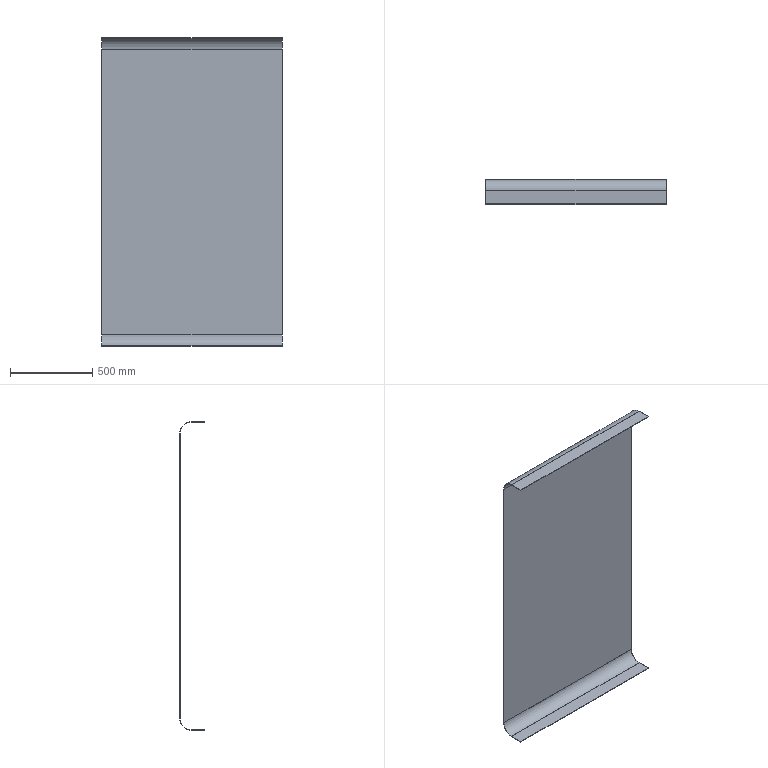Component | SolidWorks | TopHousingAssembly-1_CasingB-1 | 1 solid | 22 faces | box 1100 x 149.5 x 1881 mm | volume 6981573 mm3 | plane 18 | cylinder 4 | commonest cylinder face diameters 139 x2 133 x2
STEP:
#1=CARTESIAN_POINT('',(0.,96.791,2.618));
#2=VERTEX_POINT('',#1);
#3=CARTESIAN_POINT('',(0.,96.909,2.618));
#4=VERTEX_POINT('',#3);
#5=CARTESIAN_POINT('',(0.,96.909,2.618));
#6=DIRECTION('',(0.,1.,0.));
#7=VECTOR('',#6,39.37);
#8=LINE('',#5,#7);
#9=EDGE_CURVE('',#2,#4,#8,.T.);
#10=ORIENTED_EDGE('',*,*,#9,.F.);
#11=CARTESIAN_POINT('',(0.,96.791,71.201));
#12=VERTEX_POINT('',#11);
#13=CARTESIAN_POINT('',(0.,96.791,36.909));
#14=DIRECTION('',(0.,0.,1.));
#15=VECTOR('',#14,39.37);
#16=LINE('',#13,#15);
#17=EDGE_CURVE('',#2,#12,#16,.T.);
#18=ORIENTED_EDGE('',*,*,#17,.T.);
#19=CARTESIAN_POINT('',(0.,96.909,71.201));
#20=VERTEX_POINT('',#19);
#21=CARTESIAN_POINT('',(0.,96.909,71.201));
#22=DIRECTION('',(0.,1.,0.));
#23=VECTOR('',#22,39.37);
#24=LINE('',#21,#23);
#25=EDGE_CURVE('',#12,#20,#24,.T.);
#26=ORIENTED_EDGE('',*,*,#25,.T.);
#27=CARTESIAN_POINT('',(0.,96.909,71.201));
#28=DIRECTION('',(0.,0.,1.));
#29=VECTOR('',#28,39.37);
#30=LINE('',#27,#29);
#31=EDGE_CURVE('',#4,#20,#30,.T.);
#32=ORIENTED_EDGE('',*,*,#31,.F.);
#33=EDGE_LOOP('',(#10,#18,#26,#32));
#34=FACE_OUTER_BOUND('',#33,.T.);
#35=CARTESIAN_POINT('',(0.,96.909,71.201));
#36=DIRECTION('',(1.,0.,0.));
#37=DIRECTION('',(0.,0.,1.));
#38=AXIS2_PLACEMENT_3D('',#35,#36,#37);
#39=PLANE('',#38);
#40=ADVANCED_FACE('',(#34),#39,.F.);
#41=CARTESIAN_POINT('',(43.307,96.791,71.201));
#42=VERTEX_POINT('',#41);
#43=CARTESIAN_POINT('',(43.307,96.909,71.201));
#44=VERTEX_POINT('',#43);
#45=CARTESIAN_POINT('',(43.307,96.909,71.201));
#46=DIRECTION('',(0.,1.,0.));
#47=VECTOR('',#46,39.37);
#48=LINE('',#45,#47);
#49=EDGE_CURVE('',#42,#44,#48,.T.);
#50=ORIENTED_EDGE('',*,*,#49,.F.);
#51=CARTESIAN_POINT('',(43.307,96.791,2.618));
#52=VERTEX_POINT('',#51);
#53=CARTESIAN_POINT('',(43.307,96.791,36.909));
#54=DIRECTION('',(0.,0.,-1.));
#55=VECTOR('',#54,39.37);
#56=LINE('',#53,#55);
#57=EDGE_CURVE('',#42,#52,#56,.T.);
#58=ORIENTED_EDGE('',*,*,#57,.T.);
#59=CARTESIAN_POINT('',(43.307,96.909,2.618));
#60=VERTEX_POINT('',#59);
#61=CARTESIAN_POINT('',(43.307,96.909,2.618));
#62=DIRECTION('',(0.,1.,0.));
#63=VECTOR('',#62,39.37);
#64=LINE('',#61,#63);
#65=EDGE_CURVE('',#52,#60,#64,.T.);
#66=ORIENTED_EDGE('',*,*,#65,.T.);
#67=CARTESIAN_POINT('',(43.307,96.909,71.201));
#68=DIRECTION('',(0.,0.,-1.));
#69=VECTOR('',#68,39.37);
#70=LINE('',#67,#69);
#71=EDGE_CURVE('',#44,#60,#70,.T.);
#72=ORIENTED_EDGE('',*,*,#71,.F.);
#73=EDGE_LOOP('',(#50,#58,#66,#72));
#74=FACE_OUTER_BOUND('',#73,.T.);
#75=CARTESIAN_POINT('',(43.307,96.909,71.201));
#76=DIRECTION('',(-1.,0.,0.));
#77=DIRECTION('',(0.,0.,-1.));
#78=AXIS2_PLACEMENT_3D('',#75,#76,#77);
#79=PLANE('',#78);
#80=ADVANCED_FACE('',(#74),#79,.F.);
#81=ORIENTED_EDGE('',*,*,#71,.T.);
#82=CARTESIAN_POINT('',(0.,96.909,2.618));
#83=DIRECTION('',(-1.,0.,0.));
#84=VECTOR('',#83,39.37);
#85=LINE('',#82,#84);
#86=EDGE_CURVE('',#60,#4,#85,.T.);
#87=ORIENTED_EDGE('',*,*,#86,.T.);
#88=ORIENTED_EDGE('',*,*,#31,.T.);
#89=CARTESIAN_POINT('',(0.,96.909,71.201));
#90=DIRECTION('',(1.,0.,0.));
#91=VECTOR('',#90,39.37);
#92=LINE('',#89,#91);
#93=EDGE_CURVE('',#20,#44,#92,.T.);
#94=ORIENTED_EDGE('',*,*,#93,.T.);
#95=EDGE_LOOP('',(#81,#87,#88,#94));
#96=FACE_OUTER_BOUND('',#95,.T.);
#97=CARTESIAN_POINT('',(21.654,96.909,36.909));
#98=DIRECTION('',(0.,-1.,0.));
#99=DIRECTION('',(0.,0.,-1.));
#100=AXIS2_PLACEMENT_3D('',#97,#98,#99);
#101=PLANE('',#100);
#102=ADVANCED_FACE('',(#96),#101,.F.);
#103=ORIENTED_EDGE('',*,*,#57,.F.);
#104=CARTESIAN_POINT('',(21.654,96.791,71.201));
#105=DIRECTION('',(1.,0.,0.));
#106=VECTOR('',#105,39.37);
#107=LINE('',#104,#106);
#108=EDGE_CURVE('',#12,#42,#107,.T.);
#109=ORIENTED_EDGE('',*,*,#108,.F.);
#110=ORIENTED_EDGE('',*,*,#17,.F.);
#111=CARTESIAN_POINT('',(21.654,96.791,2.618));
#112=DIRECTION('',(-1.,0.,0.));
#113=VECTOR('',#112,39.37);
#114=LINE('',#111,#113);
#115=EDGE_CURVE('',#52,#2,#114,.T.);
#116=ORIENTED_EDGE('',*,*,#115,.F.);
#117=EDGE_LOOP('',(#103,#109,#110,#116));
#118=FACE_OUTER_BOUND('',#117,.T.);
#119=CARTESIAN_POINT('',(21.654,96.791,36.909));
#120=DIRECTION('',(0.,-1.,0.));
#121=DIRECTION('',(0.,0.,-1.));
#122=AXIS2_PLACEMENT_3D('',#119,#120,#121);
#123=PLANE('',#122);
#124=ADVANCED_FACE('',(#118),#123,.T.);
#125=CARTESIAN_POINT('',(43.307,94.173,73.819));
#126=VERTEX_POINT('',#125);
#127=CARTESIAN_POINT('',(43.307,94.173,73.937));
#128=VERTEX_POINT('',#127);
#129=CARTESIAN_POINT('',(43.307,94.173,73.937));
#130=DIRECTION('',(0.,0.,1.));
#131=VECTOR('',#130,39.37);
#132=LINE('',#129,#131);
#133=EDGE_CURVE('',#126,#128,#132,.T.);
#134=ORIENTED_EDGE('',*,*,#133,.F.);
#135=CARTESIAN_POINT('',(43.307,94.173,71.201));
#136=DIRECTION('',(1.,0.,0.));
#137=DIRECTION('',(0.,-0.,1.));
#138=AXIS2_PLACEMENT_3D('',#135,#136,#137);
#139=CIRCLE('',#138,2.618);
#140=EDGE_CURVE('',#42,#126,#139,.T.);
#141=ORIENTED_EDGE('',*,*,#140,.F.);
#142=ORIENTED_EDGE('',*,*,#49,.T.);
#143=CARTESIAN_POINT('',(43.307,94.173,71.201));
#144=DIRECTION('',(1.,0.,0.));
#145=DIRECTION('',(0.,-0.,1.));
#146=AXIS2_PLACEMENT_3D('',#143,#144,#145);
#147=CIRCLE('',#146,2.736);
#148=EDGE_CURVE('',#44,#128,#147,.T.);
#149=ORIENTED_EDGE('',*,*,#148,.T.);
#150=EDGE_LOOP('',(#134,#141,#142,#149));
#151=FACE_OUTER_BOUND('',#150,.T.);
#152=CARTESIAN_POINT('',(43.307,94.173,71.201));
#153=DIRECTION('',(1.,0.,0.));
#154=DIRECTION('',(0.,0.,-1.));
#155=AXIS2_PLACEMENT_3D('',#152,#153,#154);
#156=PLANE('',#155);
#157=ADVANCED_FACE('',(#151),#156,.T.);
#158=CARTESIAN_POINT('',(0.,94.173,73.819));
#159=VERTEX_POINT('',#158);
#160=CARTESIAN_POINT('',(0.,94.173,71.201));
#161=DIRECTION('',(-1.,0.,0.));
#162=DIRECTION('',(0.,0.,1.));
#163=AXIS2_PLACEMENT_3D('',#160,#161,#162);
#164=CIRCLE('',#163,2.618);
#165=EDGE_CURVE('',#159,#12,#164,.T.);
#166=ORIENTED_EDGE('',*,*,#165,.F.);
#167=CARTESIAN_POINT('',(0.,94.173,73.937));
#168=VERTEX_POINT('',#167);
#169=CARTESIAN_POINT('',(0.,94.173,73.819));
#170=DIRECTION('',(0.,0.,1.));
#171=VECTOR('',#170,39.37);
#172=LINE('',#169,#171);
#173=EDGE_CURVE('',#159,#168,#172,.T.);
#174=ORIENTED_EDGE('',*,*,#173,.T.);
#175=CARTESIAN_POINT('',(0.,94.173,71.201));
#176=DIRECTION('',(-1.,0.,0.));
#177=DIRECTION('',(0.,0.,1.));
#178=AXIS2_PLACEMENT_3D('',#175,#176,#177);
#179=CIRCLE('',#178,2.736);
#180=EDGE_CURVE('',#168,#20,#179,.T.);
#181=ORIENTED_EDGE('',*,*,#180,.T.);
#182=ORIENTED_EDGE('',*,*,#25,.F.);
#183=EDGE_LOOP('',(#166,#174,#181,#182));
#184=FACE_OUTER_BOUND('',#183,.T.);
#185=CARTESIAN_POINT('',(0.,94.173,71.201));
#186=DIRECTION('',(1.,0.,0.));
#187=DIRECTION('',(0.,0.,-1.));
#188=AXIS2_PLACEMENT_3D('',#185,#186,#187);
#189=PLANE('',#188);
#190=ADVANCED_FACE('',(#184),#189,.F.);
#191=ORIENTED_EDGE('',*,*,#93,.F.);
#192=ORIENTED_EDGE('',*,*,#180,.F.);
#193=CARTESIAN_POINT('',(43.307,94.173,73.937));
#194=DIRECTION('',(1.,0.,0.));
#195=VECTOR('',#194,39.37);
#196=LINE('',#193,#195);
#197=EDGE_CURVE('',#168,#128,#196,.T.);
#198=ORIENTED_EDGE('',*,*,#197,.T.);
#199=ORIENTED_EDGE('',*,*,#148,.F.);
#200=EDGE_LOOP('',(#191,#192,#198,#199));
#201=FACE_OUTER_BOUND('',#200,.T.);
#202=CARTESIAN_POINT('',(0.,94.173,71.201));
#203=DIRECTION('',(-1.,0.,0.));
#204=DIRECTION('',(0.,0.,1.));
#205=AXIS2_PLACEMENT_3D('',#202,#203,#204);
#206=CYLINDRICAL_SURFACE('',#205,2.736);
#207=ADVANCED_FACE('',(#201),#206,.T.);
#208=ORIENTED_EDGE('',*,*,#108,.T.);
#209=ORIENTED_EDGE('',*,*,#140,.T.);
#210=CARTESIAN_POINT('',(43.307,94.173,73.819));
#211=DIRECTION('',(-1.,0.,0.));
#212=VECTOR('',#211,39.37);
#213=LINE('',#210,#212);
#214=EDGE_CURVE('',#126,#159,#213,.T.);
#215=ORIENTED_EDGE('',*,*,#214,.T.);
#216=ORIENTED_EDGE('',*,*,#165,.T.);
#217=EDGE_LOOP('',(#208,#209,#215,#216));
#218=FACE_OUTER_BOUND('',#217,.T.);
#219=CARTESIAN_POINT('',(0.,94.173,71.201));
#220=DIRECTION('',(-1.,0.,0.));
#221=DIRECTION('',(0.,0.,1.));
#222=AXIS2_PLACEMENT_3D('',#219,#220,#221);
#223=CYLINDRICAL_SURFACE('',#222,2.618);
#224=ADVANCED_FACE('',(#218),#223,.F.);
#225=ORIENTED_EDGE('',*,*,#173,.F.);
#226=CARTESIAN_POINT('',(0.,91.024,73.819));
#227=VERTEX_POINT('',#226);
#228=CARTESIAN_POINT('',(0.,91.024,73.819));
#229=DIRECTION('',(0.,-1.,0.));
#230=VECTOR('',#229,39.37);
#231=LINE('',#228,#230);
#232=EDGE_CURVE('',#159,#227,#231,.T.);
#233=ORIENTED_EDGE('',*,*,#232,.T.);
#234=CARTESIAN_POINT('',(0.,91.024,73.937));
#235=VERTEX_POINT('',#234);
#236=CARTESIAN_POINT('',(0.,91.024,73.937));
#237=DIRECTION('',(0.,-0.,-1.));
#238=VECTOR('',#237,39.37);
#239=LINE('',#236,#238);
#240=EDGE_CURVE('',#235,#227,#239,.T.);
#241=ORIENTED_EDGE('',*,*,#240,.F.);
#242=CARTESIAN_POINT('',(0.,96.791,73.937));
#243=DIRECTION('',(0.,-1.,0.));
#244=VECTOR('',#243,39.37);
#245=LINE('',#242,#244);
#246=EDGE_CURVE('',#168,#235,#245,.T.);
#247=ORIENTED_EDGE('',*,*,#246,.F.);
#248=EDGE_LOOP('',(#225,#233,#241,#247));
#249=FACE_OUTER_BOUND('',#248,.T.);
#250=CARTESIAN_POINT('',(0.,91.024,73.937));
#251=DIRECTION('',(1.,0.,-0.));
#252=DIRECTION('',(-0.,1.,0.));
#253=AXIS2_PLACEMENT_3D('',#250,#251,#252);
#254=PLANE('',#253);
#255=ADVANCED_FACE('',(#249),#254,.F.);
#256=ORIENTED_EDGE('',*,*,#133,.T.);
#257=CARTESIAN_POINT('',(43.307,91.024,73.937));
#258=VERTEX_POINT('',#257);
#259=CARTESIAN_POINT('',(43.307,96.791,73.937));
#260=DIRECTION('',(0.,1.,-0.));
#261=VECTOR('',#260,39.37);
#262=LINE('',#259,#261);
#263=EDGE_CURVE('',#258,#128,#262,.T.);
#264=ORIENTED_EDGE('',*,*,#263,.F.);
#265=CARTESIAN_POINT('',(43.307,91.024,73.819));
#266=VERTEX_POINT('',#265);
#267=CARTESIAN_POINT('',(43.307,91.024,73.937));
#268=DIRECTION('',(0.,-0.,-1.));
#269=VECTOR('',#268,39.37);
#270=LINE('',#267,#269);
#271=EDGE_CURVE('',#258,#266,#270,.T.);
#272=ORIENTED_EDGE('',*,*,#271,.T.);
#273=CARTESIAN_POINT('',(43.307,96.791,73.819));
#274=DIRECTION('',(0.,1.,-0.));
#275=VECTOR('',#274,39.37);
#276=LINE('',#273,#275);
#277=EDGE_CURVE('',#266,#126,#276,.T.);
#278=ORIENTED_EDGE('',*,*,#277,.T.);
#279=EDGE_LOOP('',(#256,#264,#272,#278));
#280=FACE_OUTER_BOUND('',#279,.T.);
#281=CARTESIAN_POINT('',(43.307,96.791,73.937));
#282=DIRECTION('',(-1.,0.,0.));
#283=DIRECTION('',(0.,0.,1.));
#284=AXIS2_PLACEMENT_3D('',#281,#282,#283);
#285=PLANE('',#284);
#286=ADVANCED_FACE('',(#280),#285,.F.);
#287=ORIENTED_EDGE('',*,*,#197,.F.);
#288=ORIENTED_EDGE('',*,*,#246,.T.);
#289=CARTESIAN_POINT('',(21.654,91.024,73.937));
#290=DIRECTION('',(1.,0.,0.));
#291=VECTOR('',#290,39.37);
#292=LINE('',#289,#291);
#293=EDGE_CURVE('',#235,#258,#292,.T.);
#294=ORIENTED_EDGE('',*,*,#293,.T.);
#295=ORIENTED_EDGE('',*,*,#263,.T.);
#296=EDGE_LOOP('',(#287,#288,#294,#295));
#297=FACE_OUTER_BOUND('',#296,.T.);
#298=CARTESIAN_POINT('',(21.654,96.791,73.937));
#299=DIRECTION('',(0.,-0.,-1.));
#300=DIRECTION('',(0.,1.,-0.));
#301=AXIS2_PLACEMENT_3D('',#298,#299,#300);
#302=PLANE('',#301);
#303=ADVANCED_FACE('',(#297),#302,.F.);
#304=ORIENTED_EDGE('',*,*,#232,.F.);
#305=ORIENTED_EDGE('',*,*,#214,.F.);
#306=ORIENTED_EDGE('',*,*,#277,.F.);
#307=CARTESIAN_POINT('',(43.307,91.024,73.819));
#308=DIRECTION('',(1.,0.,0.));
#309=VECTOR('',#308,39.37);
#310=LINE('',#307,#309);
#311=EDGE_CURVE('',#227,#266,#310,.T.);
#312=ORIENTED_EDGE('',*,*,#311,.F.);
#313=EDGE_LOOP('',(#304,#305,#306,#312));
#314=FACE_OUTER_BOUND('',#313,.T.);
#315=CARTESIAN_POINT('',(21.654,96.791,73.819));
#316=DIRECTION('',(0.,-0.,-1.));
#317=DIRECTION('',(0.,1.,-0.));
#318=AXIS2_PLACEMENT_3D('',#315,#316,#317);
#319=PLANE('',#318);
#320=ADVANCED_FACE('',(#314),#319,.T.);
#321=ORIENTED_EDGE('',*,*,#311,.T.);
#322=ORIENTED_EDGE('',*,*,#271,.F.);
#323=ORIENTED_EDGE('',*,*,#293,.F.);
#324=ORIENTED_EDGE('',*,*,#240,.T.);
#325=EDGE_LOOP('',(#321,#322,#323,#324));
#326=FACE_OUTER_BOUND('',#325,.T.);
#327=CARTESIAN_POINT('',(43.307,91.024,73.937));
#328=DIRECTION('',(0.,1.,-0.));
#329=DIRECTION('',(0.,0.,1.));
#330=AXIS2_PLACEMENT_3D('',#327,#328,#329);
#331=PLANE('',#330);
#332=ADVANCED_FACE('',(#326),#331,.F.);
#333=CARTESIAN_POINT('',(0.,94.173,-0.));
#334=VERTEX_POINT('',#333);
#335=CARTESIAN_POINT('',(0.,94.173,-0.1181));
#336=VERTEX_POINT('',#335);
#337=CARTESIAN_POINT('',(0.,94.173,-0.1181));
#338=DIRECTION('',(0.,0.,-1.));
#339=VECTOR('',#338,39.37);
#340=LINE('',#337,#339);
#341=EDGE_CURVE('',#334,#336,#340,.T.);
#342=ORIENTED_EDGE('',*,*,#341,.F.);
#343=CARTESIAN_POINT('',(0.,94.173,2.618));
#344=DIRECTION('',(-1.,0.,0.));
#345=DIRECTION('',(0.,-0.,-1.));
#346=AXIS2_PLACEMENT_3D('',#343,#344,#345);
#347=CIRCLE('',#346,2.618);
#348=EDGE_CURVE('',#2,#334,#347,.T.);
#349=ORIENTED_EDGE('',*,*,#348,.F.);
#350=ORIENTED_EDGE('',*,*,#9,.T.);
#351=CARTESIAN_POINT('',(0.,94.173,2.618));
#352=DIRECTION('',(-1.,0.,0.));
#353=DIRECTION('',(0.,-0.,-1.));
#354=AXIS2_PLACEMENT_3D('',#351,#352,#353);
#355=CIRCLE('',#354,2.736);
#356=EDGE_CURVE('',#4,#336,#355,.T.);
#357=ORIENTED_EDGE('',*,*,#356,.T.);
#358=EDGE_LOOP('',(#342,#349,#350,#357));
#359=FACE_OUTER_BOUND('',#358,.T.);
#360=CARTESIAN_POINT('',(0.,94.173,2.618));
#361=DIRECTION('',(-1.,0.,0.));
#362=DIRECTION('',(0.,0.,1.));
#363=AXIS2_PLACEMENT_3D('',#360,#361,#362);
#364=PLANE('',#363);
#365=ADVANCED_FACE('',(#359),#364,.T.);
#366=CARTESIAN_POINT('',(43.307,94.173,-0.));
#367=VERTEX_POINT('',#366);
#368=CARTESIAN_POINT('',(43.307,94.173,2.618));
#369=DIRECTION('',(1.,0.,0.));
#370=DIRECTION('',(0.,0.,-1.));
#371=AXIS2_PLACEMENT_3D('',#368,#369,#370);
#372=CIRCLE('',#371,2.618);
#373=EDGE_CURVE('',#367,#52,#372,.T.);
#374=ORIENTED_EDGE('',*,*,#373,.F.);
#375=CARTESIAN_POINT('',(43.307,94.173,-0.1181));
#376=VERTEX_POINT('',#375);
#377=CARTESIAN_POINT('',(43.307,94.173,-0.));
#378=DIRECTION('',(-0.,0.,-1.));
#379=VECTOR('',#378,39.37);
#380=LINE('',#377,#379);
#381=EDGE_CURVE('',#367,#376,#380,.T.);
#382=ORIENTED_EDGE('',*,*,#381,.T.);
#383=CARTESIAN_POINT('',(43.307,94.173,2.618));
#384=DIRECTION('',(1.,0.,0.));
#385=DIRECTION('',(0.,0.,-1.));
#386=AXIS2_PLACEMENT_3D('',#383,#384,#385);
#387=CIRCLE('',#386,2.736);
#388=EDGE_CURVE('',#376,#60,#387,.T.);
#389=ORIENTED_EDGE('',*,*,#388,.T.);
#390=ORIENTED_EDGE('',*,*,#65,.F.);
#391=EDGE_LOOP('',(#374,#382,#389,#390));
#392=FACE_OUTER_BOUND('',#391,.T.);
#393=CARTESIAN_POINT('',(43.307,94.173,2.618));
#394=DIRECTION('',(-1.,0.,0.));
#395=DIRECTION('',(0.,0.,1.));
#396=AXIS2_PLACEMENT_3D('',#393,#394,#395);
#397=PLANE('',#396);
#398=ADVANCED_FACE('',(#392),#397,.F.);
#399=ORIENTED_EDGE('',*,*,#86,.F.);
#400=ORIENTED_EDGE('',*,*,#388,.F.);
#401=CARTESIAN_POINT('',(0.,94.173,-0.1181));
#402=DIRECTION('',(-1.,0.,0.));
#403=VECTOR('',#402,39.37);
#404=LINE('',#401,#403);
#405=EDGE_CURVE('',#376,#336,#404,.T.);
#406=ORIENTED_EDGE('',*,*,#405,.T.);
#407=ORIENTED_EDGE('',*,*,#356,.F.);
#408=EDGE_LOOP('',(#399,#400,#406,#407));
#409=FACE_OUTER_BOUND('',#408,.T.);
#410=CARTESIAN_POINT('',(43.307,94.173,2.618));
#411=DIRECTION('',(1.,0.,0.));
#412=DIRECTION('',(0.,0.,-1.));
#413=AXIS2_PLACEMENT_3D('',#410,#411,#412);
#414=CYLINDRICAL_SURFACE('',#413,2.736);
#415=ADVANCED_FACE('',(#409),#414,.T.);
#416=ORIENTED_EDGE('',*,*,#115,.T.);
#417=ORIENTED_EDGE('',*,*,#348,.T.);
#418=CARTESIAN_POINT('',(0.,94.173,-0.));
#419=DIRECTION('',(1.,0.,0.));
#420=VECTOR('',#419,39.37);
#421=LINE('',#418,#420);
#422=EDGE_CURVE('',#334,#367,#421,.T.);
#423=ORIENTED_EDGE('',*,*,#422,.T.);
#424=ORIENTED_EDGE('',*,*,#373,.T.);
#425=EDGE_LOOP('',(#416,#417,#423,#424));
#426=FACE_OUTER_BOUND('',#425,.T.);
#427=CARTESIAN_POINT('',(43.307,94.173,2.618));
#428=DIRECTION('',(1.,0.,0.));
#429=DIRECTION('',(0.,0.,-1.));
#430=AXIS2_PLACEMENT_3D('',#427,#428,#429);
#431=CYLINDRICAL_SURFACE('',#430,2.618);
#432=ADVANCED_FACE('',(#426),#431,.F.);
#433=ORIENTED_EDGE('',*,*,#381,.F.);
#434=CARTESIAN_POINT('',(43.307,91.024,-0.));
#435=VERTEX_POINT('',#434);
#436=CARTESIAN_POINT('',(43.307,91.024,-0.));
#437=DIRECTION('',(0.,-1.,-0.));
#438=VECTOR('',#437,39.37);
#439=LINE('',#436,#438);
#440=EDGE_CURVE('',#367,#435,#439,.T.);
#441=ORIENTED_EDGE('',*,*,#440,.T.);
#442=CARTESIAN_POINT('',(43.307,91.024,-0.1181));
#443=VERTEX_POINT('',#442);
#444=CARTESIAN_POINT('',(43.307,91.024,-0.1181));
#445=DIRECTION('',(0.,-0.,1.));
#446=VECTOR('',#445,39.37);
#447=LINE('',#444,#446);
#448=EDGE_CURVE('',#443,#435,#447,.T.);
#449=ORIENTED_EDGE('',*,*,#448,.F.);
#450=CARTESIAN_POINT('',(43.307,96.791,-0.1181));
#451=DIRECTION('',(0.,-1.,-0.));
#452=VECTOR('',#451,39.37);
#453=LINE('',#450,#452);
#454=EDGE_CURVE('',#376,#443,#453,.T.);
#455=ORIENTED_EDGE('',*,*,#454,.F.);
#456=EDGE_LOOP('',(#433,#441,#449,#455));
#457=FACE_OUTER_BOUND('',#456,.T.);
#458=CARTESIAN_POINT('',(43.307,91.024,-0.1181));
#459=DIRECTION('',(-1.,-0.,-0.));
#460=DIRECTION('',(0.,-1.,0.));
#461=AXIS2_PLACEMENT_3D('',#458,#459,#460);
#462=PLANE('',#461);
#463=ADVANCED_FACE('',(#457),#462,.F.);
#464=ORIENTED_EDGE('',*,*,#341,.T.);
#465=CARTESIAN_POINT('',(0.,91.024,-0.1181));
#466=VERTEX_POINT('',#465);
#467=CARTESIAN_POINT('',(0.,96.791,-0.1181));
#468=DIRECTION('',(0.,1.,0.));
#469=VECTOR('',#468,39.37);
#470=LINE('',#467,#469);
#471=EDGE_CURVE('',#466,#336,#470,.T.);
#472=ORIENTED_EDGE('',*,*,#471,.F.);
#473=CARTESIAN_POINT('',(0.,91.024,-0.));
#474=VERTEX_POINT('',#473);
#475=CARTESIAN_POINT('',(0.,91.024,-0.1181));
#476=DIRECTION('',(0.,-0.,1.));
#477=VECTOR('',#476,39.37);
#478=LINE('',#475,#477);
#479=EDGE_CURVE('',#466,#474,#478,.T.);
#480=ORIENTED_EDGE('',*,*,#479,.T.);
#481=CARTESIAN_POINT('',(0.,96.791,-0.));
#482=DIRECTION('',(0.,1.,0.));
#483=VECTOR('',#482,39.37);
#484=LINE('',#481,#483);
#485=EDGE_CURVE('',#474,#334,#484,.T.);
#486=ORIENTED_EDGE('',*,*,#485,.T.);
#487=EDGE_LOOP('',(#464,#472,#480,#486));
#488=FACE_OUTER_BOUND('',#487,.T.);
#489=CARTESIAN_POINT('',(0.,96.791,-0.1181));
#490=DIRECTION('',(1.,0.,0.));
#491=DIRECTION('',(0.,0.,-1.));
#492=AXIS2_PLACEMENT_3D('',#489,#490,#491);
#493=PLANE('',#492);
#494=ADVANCED_FACE('',(#488),#493,.F.);
#495=ORIENTED_EDGE('',*,*,#405,.F.);
#496=ORIENTED_EDGE('',*,*,#454,.T.);
#497=CARTESIAN_POINT('',(21.654,91.024,-0.1181));
#498=DIRECTION('',(-1.,0.,0.));
#499=VECTOR('',#498,39.37);
#500=LINE('',#497,#499);
#501=EDGE_CURVE('',#443,#466,#500,.T.);
#502=ORIENTED_EDGE('',*,*,#501,.T.);
#503=ORIENTED_EDGE('',*,*,#471,.T.);
#504=EDGE_LOOP('',(#495,#496,#502,#503));
#505=FACE_OUTER_BOUND('',#504,.T.);
#506=CARTESIAN_POINT('',(21.654,96.791,-0.1181));
#507=DIRECTION('',(0.,-0.,1.));
#508=DIRECTION('',(0.,-1.,-0.));
#509=AXIS2_PLACEMENT_3D('',#506,#507,#508);
#510=PLANE('',#509);
#511=ADVANCED_FACE('',(#505),#510,.F.);
#512=ORIENTED_EDGE('',*,*,#440,.F.);
#513=ORIENTED_EDGE('',*,*,#422,.F.);
#514=ORIENTED_EDGE('',*,*,#485,.F.);
#515=CARTESIAN_POINT('',(0.,91.024,-0.));
#516=DIRECTION('',(-1.,0.,0.));
#517=VECTOR('',#516,39.37);
#518=LINE('',#515,#517);
#519=EDGE_CURVE('',#435,#474,#518,.T.);
#520=ORIENTED_EDGE('',*,*,#519,.F.);
#521=EDGE_LOOP('',(#512,#513,#514,#520));
#522=FACE_OUTER_BOUND('',#521,.T.);
#523=CARTESIAN_POINT('',(21.654,96.791,-0.));
#524=DIRECTION('',(0.,-0.,1.));
#525=DIRECTION('',(0.,-1.,-0.));
#526=AXIS2_PLACEMENT_3D('',#523,#524,#525);
#527=PLANE('',#526);
#528=ADVANCED_FACE('',(#522),#527,.T.);
#529=ORIENTED_EDGE('',*,*,#519,.T.);
#530=ORIENTED_EDGE('',*,*,#479,.F.);
#531=ORIENTED_EDGE('',*,*,#501,.F.);
#532=ORIENTED_EDGE('',*,*,#448,.T.);
#533=EDGE_LOOP('',(#529,#530,#531,#532));
#534=FACE_OUTER_BOUND('',#533,.T.);
#535=CARTESIAN_POINT('',(0.,91.024,-0.1181));
#536=DIRECTION('',(0.,1.,0.));
#537=DIRECTION('',(0.,-0.,1.));
#538=AXIS2_PLACEMENT_3D('',#535,#536,#537);
#539=PLANE('',#538);
#540=ADVANCED_FACE('',(#534),#539,.F.);
#541=CLOSED_SHELL('',(#40,#80,#102,#124,#157,#190,#207,#224,#255,#286,#303,#320,#332,#365,#398,#415,#432,#463,#494,#511,#528,#540));
#542=MANIFOLD_SOLID_BREP('',#541);
#543=CARTESIAN_POINT('',(0.,0.,0.));
#544=DIRECTION('',(0.,0.,1.));
#545=DIRECTION('',(1.,0.,0.));
#546=AXIS2_PLACEMENT_3D('',#543,#544,#545);
#547=(LENGTH_UNIT()NAMED_UNIT(*)SI_UNIT($,.METRE.));
#548=LENGTH_MEASURE_WITH_UNIT(LENGTH_MEASURE(0.0254),#547);
#549=DIMENSIONAL_EXPONENTS(1.,0.,0.,0.,0.,0.,0.);
#550=(CONVERSION_BASED_UNIT('',#548)LENGTH_UNIT()NAMED_UNIT(#549));
#551=UNCERTAINTY_MEASURE_WITH_UNIT(LENGTH_MEASURE(0.00001),#550,'','');
#552=(NAMED_UNIT(*)PLANE_ANGLE_UNIT()SI_UNIT($,.RADIAN.));
#553=(NAMED_UNIT(*)SI_UNIT($,.STERADIAN.)SOLID_ANGLE_UNIT());
#554=(GEOMETRIC_REPRESENTATION_CONTEXT(3)GLOBAL_UNCERTAINTY_ASSIGNED_CONTEXT((#551))GLOBAL_UNIT_ASSIGNED_CONTEXT((#550,#552,#553))REPRESENTATION_CONTEXT('',''));
#555=ADVANCED_BREP_SHAPE_REPRESENTATION('',(#542,#546),#554);
#556=COLOUR_RGB('',0.7922,0.8196,0.9333);
#557=FILL_AREA_STYLE_COLOUR('',#556);
#558=FILL_AREA_STYLE('',(#557));
#559=SURFACE_STYLE_FILL_AREA(#558);
#560=SURFACE_SIDE_STYLE('',(#559));
#561=SURFACE_STYLE_USAGE(.BOTH.,#560);
#562=PRESENTATION_STYLE_ASSIGNMENT((#561));
#563=STYLED_ITEM('',(#562),#542);
#564=PRESENTATION_LAYER_ASSIGNMENT('','',(#563));
#565=(LENGTH_UNIT()NAMED_UNIT(*)SI_UNIT($,.METRE.));
#566=LENGTH_MEASURE_WITH_UNIT(LENGTH_MEASURE(0.0254),#565);
#567=DIMENSIONAL_EXPONENTS(1.,0.,0.,0.,0.,0.,0.);
#568=(CONVERSION_BASED_UNIT('',#566)LENGTH_UNIT()NAMED_UNIT(#567));
#569=UNCERTAINTY_MEASURE_WITH_UNIT(LENGTH_MEASURE(0.00001),#568,'','');
#570=(NAMED_UNIT(*)PLANE_ANGLE_UNIT()SI_UNIT($,.RADIAN.));
#571=(NAMED_UNIT(*)SI_UNIT($,.STERADIAN.)SOLID_ANGLE_UNIT());
#572=(GEOMETRIC_REPRESENTATION_CONTEXT(3)GLOBAL_UNCERTAINTY_ASSIGNED_CONTEXT((#569))GLOBAL_UNIT_ASSIGNED_CONTEXT((#568,#570,#571))REPRESENTATION_CONTEXT('',''));
#573=MECHANICAL_DESIGN_GEOMETRIC_PRESENTATION_REPRESENTATION('',(#563),#572);